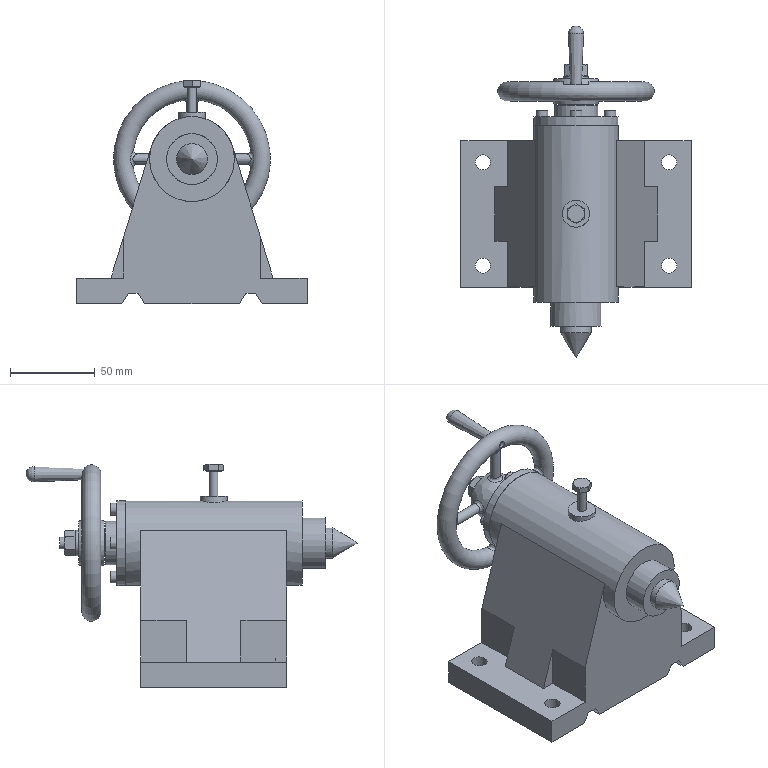Assembly | NX | mm | 15 component files | 15 solids | 292 faces | box 135.6 x 195.41 x 131.4 mm | volume 541191 mm3 | plane 156 | cone 61 | cylinder 55 | torus 10 | spline 9 | sphere 1 | commonest cylinder face diameters 3.3 x8 3 x4 7 x4 6 x4 4.5 x4 9 x4 11.3 x2 10.3 x2
Bill of materials:
GB-T5782-2000,M6x30 | 1 |  | Hexagon Head Bolt, GB-T 5782-2000,M6x30
unnamed part 1 | 1 |  | Solid round pin, turned shape: a conical point at one end, a long main body that tapers slightly, and a short, smaller-diameter cylindrical stub at the other end.
unnamed part 2 | 1 |  | Solid flat block with an obround outline (rounded ends): two flat parallel faces, straight sides and fully rounded ends.
unnamed part 3 | 1 |  | Solid stepped round shaft: a long plain section on one side of a raised collar, then several steps of decreasing diameter on the other side. One stepped section has an elongated slot with rounded ends.
unnamed part 4 | 1 |  | Spoked wheel: a rim with a round cross-section (like a ring), four straight round spokes at 90 degrees, and a central hub with a through bore. The bore has a small rectangular notch. There is a small round hole through the rim.
unnamed part 5 | 1 |  | Hollow cylindrical sleeve (tube) with a straight through bore and a shallow flat cut into part of its outer surface, partway along its length.
GB-T6170_F-2000,M8x1.25 | 1 |  | Hexagonal nut shape: a hex prism with a central round hole and chamfered corners on both faces.
GB-T848-2002,M8 | 1 |  | Flat annular ring (plain washer-like disc): thin circular plate with a concentric through-hole, flat parallel faces and straight cylindrical outer and inner edges.
unnamed part 6 | 1 |  | Housing on a base, similar to a pillow block: a horizontal cylindrical barrel with a through bore, held up by a tapered support on a rectangular base plate. The base has four through holes in its outer flanges. A small raised boss with a small hole sits on top of the barrel.
unnamed part 7 | 1 |  | Solid round handle-like part: a tapered body with a rounded end, and a short, smaller-diameter cylindrical spigot at the narrow end.
GB-T70.1-2000,M4x10 | 4 |  | Hexagon Socket Head Cap Screw, GB-T 70.1-2000,M4x10
unnamed part 8 | 1 |  | Round flange: a flat disc with four evenly spaced bolt-type holes, a raised round hub on one face, and a central through bore.
Mates:
1. concentric | flat_key 1 edge | screw_rod 1 edge
2. concentric | turntable 1 edge | screw_rod 1 edge
3. concentric | end_cap 1 edge | screw_rod 1 edge
4. concentric | handle 1 edge | turntable 1 arc
5. touch align | live_center 1 face | screw_sleeve 1 face
6. touch align | live_center 1 face | screw_sleeve 1 edge
7. touch align | screw_sleeve 1 face | tailstock 1 face
8. distance | screw_sleeve 1 face | tailstock 1 face
9. concentric | end_cap 1 edge | tailstock 1 edge
10. concentric | washer 1 edge | turntable 1 edge
11. concentric | nut_M8 1 edge | washer 1 edge
12. bond | end_cap 1 component | assembly component
13. bond | screw_M4x10 4 component | assembly component
14. bond | screw_M4x10 3 component | assembly component
15. bond | screw_M4x10 2 component | assembly component
16. circular | assembly datumaxis | assembly cartesiancoordinatesystem | assembly cartesiancoordinatesystem | assembly cartesiancoordinatesystem | assembly cartesiancoordinatesystem
17. bond | screw_M4x10 1 component | assembly component
18. touch align | bolt_M6x30 1 face | tailstock 1 face
19. touch align | bolt_M6x30 1 face | screw_sleeve 1 face